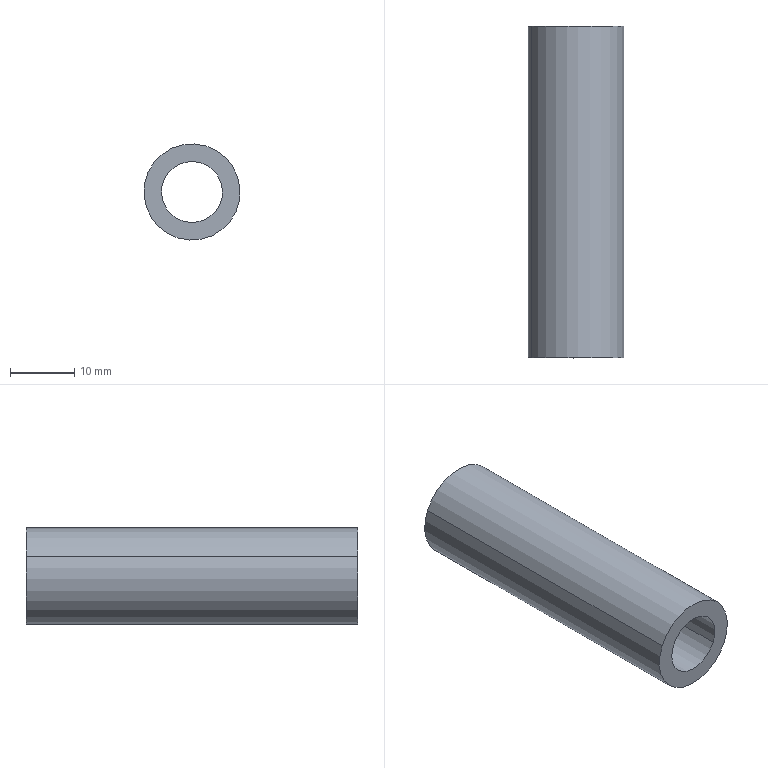Component | SolidWorks | MotorShaftHousing2-2 | 1 solid | 6 faces | box 15 x 51.75 x 15 mm | volume 5477 mm3 | cylinder 4 | plane 2 | commonest cylinder face diameters 9.5 x2 15 x2
build123d program:
from build123d import *

# Parameters (mm, degrees)
SKETCH1_R           = 7.5
SKETCH1_R_2         = 4.75
BOSS_EXTRUDE1_DEPTH = 51.75


with BuildPart() as part:
    # Sketch1 → Boss-Extrude1 (new body)
    with BuildSketch(Plane.XY):
        with Locations((-255.265, -5.179)):
            Circle(SKETCH1_R)
        with Locations((-255.265, -5.179)):
            Circle(SKETCH1_R_2, mode=Mode.SUBTRACT)
    extrude(amount=BOSS_EXTRUDE1_DEPTH)


solid = part.part

# Placed as in the assembly
solid = solid.moved(Location((218.265, 246.75, 11.179), (90, 0, 0)))
STEP:
#1=COLOUR_RGB('',0.7922,0.8196,0.9333);
#2=FILL_AREA_STYLE_COLOUR('',#1);
#3=FILL_AREA_STYLE('',(#2));
#4=SURFACE_STYLE_FILL_AREA(#3);
#5=SURFACE_SIDE_STYLE('',(#4));
#6=SURFACE_STYLE_USAGE(.BOTH.,#5);
#7=PRESENTATION_STYLE_ASSIGNMENT((#6));
#8=CARTESIAN_POINT('',(-1.628,9.715,0.3115));
#9=VERTEX_POINT('',#8);
#10=CARTESIAN_POINT('',(-1.285,9.715,0.161));
#11=VERTEX_POINT('',#10);
#12=CARTESIAN_POINT('',(-1.457,9.715,0.2362));
#13=DIRECTION('',(-0.,1.,0.));
#14=DIRECTION('',(0.9155,0.,-0.4024));
#15=AXIS2_PLACEMENT_3D('',#12,#13,#14);
#16=CIRCLE('',#15,0.187);
#17=EDGE_CURVE('',#9,#11,#16,.T.);
#18=ORIENTED_EDGE('',*,*,#17,.T.);
#19=CARTESIAN_POINT('',(-1.285,7.677,0.161));
#20=VERTEX_POINT('',#19);
#21=CARTESIAN_POINT('',(-1.285,10.55,0.161));
#22=DIRECTION('',(0.,-1.,0.));
#23=VECTOR('',#22,39.37);
#24=LINE('',#21,#23);
#25=EDGE_CURVE('',#11,#20,#24,.T.);
#26=ORIENTED_EDGE('',*,*,#25,.T.);
#27=CARTESIAN_POINT('',(-1.628,7.677,0.3115));
#28=VERTEX_POINT('',#27);
#29=CARTESIAN_POINT('',(-1.457,7.677,0.2362));
#30=DIRECTION('',(0.,1.,0.));
#31=DIRECTION('',(0.9155,0.,-0.4024));
#32=AXIS2_PLACEMENT_3D('',#29,#30,#31);
#33=CIRCLE('',#32,0.187);
#34=EDGE_CURVE('',#28,#20,#33,.T.);
#35=ORIENTED_EDGE('',*,*,#34,.F.);
#36=CARTESIAN_POINT('',(-1.628,10.55,0.3115));
#37=DIRECTION('',(0.,-1.,0.));
#38=VECTOR('',#37,39.37);
#39=LINE('',#36,#38);
#40=EDGE_CURVE('',#9,#28,#39,.T.);
#41=ORIENTED_EDGE('',*,*,#40,.F.);
#42=EDGE_LOOP('',(#18,#26,#35,#41));
#43=FACE_OUTER_BOUND('',#42,.T.);
#44=CARTESIAN_POINT('',(-1.457,10.55,0.2362));
#45=DIRECTION('',(0.,-1.,0.));
#46=DIRECTION('',(-0.9155,0.,0.4024));
#47=AXIS2_PLACEMENT_3D('',#44,#45,#46);
#48=CYLINDRICAL_SURFACE('',#47,0.187);
#49=ADVANCED_FACE('',(#43),#48,.F.);
#50=CARTESIAN_POINT('',(-1.186,9.715,0.1174));
#51=VERTEX_POINT('',#50);
#52=CARTESIAN_POINT('',(-1.727,9.715,0.355));
#53=VERTEX_POINT('',#52);
#54=CARTESIAN_POINT('',(-1.457,9.715,0.2362));
#55=DIRECTION('',(-0.,1.,0.));
#56=DIRECTION('',(0.9155,0.,-0.4024));
#57=AXIS2_PLACEMENT_3D('',#54,#55,#56);
#58=CIRCLE('',#57,0.2953);
#59=EDGE_CURVE('',#51,#53,#58,.T.);
#60=ORIENTED_EDGE('',*,*,#59,.F.);
#61=CARTESIAN_POINT('',(-1.186,7.677,0.1174));
#62=VERTEX_POINT('',#61);
#63=CARTESIAN_POINT('',(-1.186,10.55,0.1174));
#64=DIRECTION('',(0.,-1.,0.));
#65=VECTOR('',#64,39.37);
#66=LINE('',#63,#65);
#67=EDGE_CURVE('',#51,#62,#66,.T.);
#68=ORIENTED_EDGE('',*,*,#67,.T.);
#69=CARTESIAN_POINT('',(-1.727,7.677,0.355));
#70=VERTEX_POINT('',#69);
#71=CARTESIAN_POINT('',(-1.457,7.677,0.2362));
#72=DIRECTION('',(0.,1.,0.));
#73=DIRECTION('',(0.9155,0.,-0.4024));
#74=AXIS2_PLACEMENT_3D('',#71,#72,#73);
#75=CIRCLE('',#74,0.2953);
#76=EDGE_CURVE('',#62,#70,#75,.T.);
#77=ORIENTED_EDGE('',*,*,#76,.T.);
#78=CARTESIAN_POINT('',(-1.727,10.55,0.355));
#79=DIRECTION('',(0.,-1.,0.));
#80=VECTOR('',#79,39.37);
#81=LINE('',#78,#80);
#82=EDGE_CURVE('',#53,#70,#81,.T.);
#83=ORIENTED_EDGE('',*,*,#82,.F.);
#84=EDGE_LOOP('',(#60,#68,#77,#83));
#85=FACE_OUTER_BOUND('',#84,.T.);
#86=CARTESIAN_POINT('',(-1.457,10.55,0.2362));
#87=DIRECTION('',(0.,-1.,0.));
#88=DIRECTION('',(-0.9155,0.,0.4024));
#89=AXIS2_PLACEMENT_3D('',#86,#87,#88);
#90=CYLINDRICAL_SURFACE('',#89,0.2953);
#91=ADVANCED_FACE('',(#85),#90,.T.);
#92=ORIENTED_EDGE('',*,*,#67,.F.);
#93=CARTESIAN_POINT('',(-1.457,9.715,0.2362));
#94=DIRECTION('',(-0.,1.,0.));
#95=DIRECTION('',(0.9155,0.,-0.4024));
#96=AXIS2_PLACEMENT_3D('',#93,#94,#95);
#97=CIRCLE('',#96,0.2953);
#98=EDGE_CURVE('',#53,#51,#97,.T.);
#99=ORIENTED_EDGE('',*,*,#98,.F.);
#100=ORIENTED_EDGE('',*,*,#82,.T.);
#101=CARTESIAN_POINT('',(-1.457,7.677,0.2362));
#102=DIRECTION('',(0.,1.,0.));
#103=DIRECTION('',(0.9155,0.,-0.4024));
#104=AXIS2_PLACEMENT_3D('',#101,#102,#103);
#105=CIRCLE('',#104,0.2953);
#106=EDGE_CURVE('',#70,#62,#105,.T.);
#107=ORIENTED_EDGE('',*,*,#106,.T.);
#108=EDGE_LOOP('',(#92,#99,#100,#107));
#109=FACE_OUTER_BOUND('',#108,.T.);
#110=CARTESIAN_POINT('',(-1.457,10.55,0.2362));
#111=DIRECTION('',(0.,-1.,0.));
#112=DIRECTION('',(-0.9155,0.,0.4024));
#113=AXIS2_PLACEMENT_3D('',#110,#111,#112);
#114=CYLINDRICAL_SURFACE('',#113,0.2953);
#115=ADVANCED_FACE('',(#109),#114,.T.);
#116=ORIENTED_EDGE('',*,*,#106,.F.);
#117=ORIENTED_EDGE('',*,*,#76,.F.);
#118=EDGE_LOOP('',(#116,#117));
#119=FACE_OUTER_BOUND('',#118,.T.);
#120=ORIENTED_EDGE('',*,*,#34,.T.);
#121=CARTESIAN_POINT('',(-1.457,7.677,0.2362));
#122=DIRECTION('',(0.,1.,0.));
#123=DIRECTION('',(0.9155,0.,-0.4024));
#124=AXIS2_PLACEMENT_3D('',#121,#122,#123);
#125=CIRCLE('',#124,0.187);
#126=EDGE_CURVE('',#20,#28,#125,.T.);
#127=ORIENTED_EDGE('',*,*,#126,.T.);
#128=EDGE_LOOP('',(#120,#127));
#129=FACE_BOUND('',#128,.T.);
#130=CARTESIAN_POINT('',(-1.457,7.677,0.2362));
#131=DIRECTION('',(0.,1.,0.));
#132=DIRECTION('',(0.9155,0.,-0.4024));
#133=AXIS2_PLACEMENT_3D('',#130,#131,#132);
#134=PLANE('',#133);
#135=ADVANCED_FACE('',(#119,#129),#134,.F.);
#136=ORIENTED_EDGE('',*,*,#25,.F.);
#137=CARTESIAN_POINT('',(-1.457,9.715,0.2362));
#138=DIRECTION('',(-0.,1.,0.));
#139=DIRECTION('',(0.9155,0.,-0.4024));
#140=AXIS2_PLACEMENT_3D('',#137,#138,#139);
#141=CIRCLE('',#140,0.187);
#142=EDGE_CURVE('',#11,#9,#141,.T.);
#143=ORIENTED_EDGE('',*,*,#142,.T.);
#144=ORIENTED_EDGE('',*,*,#40,.T.);
#145=ORIENTED_EDGE('',*,*,#126,.F.);
#146=EDGE_LOOP('',(#136,#143,#144,#145));
#147=FACE_OUTER_BOUND('',#146,.T.);
#148=CARTESIAN_POINT('',(-1.457,10.55,0.2362));
#149=DIRECTION('',(0.,-1.,0.));
#150=DIRECTION('',(-0.9155,0.,0.4024));
#151=AXIS2_PLACEMENT_3D('',#148,#149,#150);
#152=CYLINDRICAL_SURFACE('',#151,0.187);
#153=ADVANCED_FACE('',(#147),#152,.F.);
#154=ORIENTED_EDGE('',*,*,#17,.F.);
#155=ORIENTED_EDGE('',*,*,#142,.F.);
#156=EDGE_LOOP('',(#154,#155));
#157=FACE_BOUND('',#156,.T.);
#158=ORIENTED_EDGE('',*,*,#98,.T.);
#159=ORIENTED_EDGE('',*,*,#59,.T.);
#160=EDGE_LOOP('',(#158,#159));
#161=FACE_OUTER_BOUND('',#160,.T.);
#162=CARTESIAN_POINT('',(-1.158,9.715,0.3643));
#163=DIRECTION('',(-0.,1.,0.));
#164=DIRECTION('',(-0.3942,-0.,0.919));
#165=AXIS2_PLACEMENT_3D('',#162,#163,#164);
#166=PLANE('',#165);
#167=ADVANCED_FACE('',(#157,#161),#166,.T.);
#168=CLOSED_SHELL('',(#49,#91,#115,#135,#153,#167));
#169=MANIFOLD_SOLID_BREP('',#168);
#170=STYLED_ITEM('',(#7),#169);
#171=(LENGTH_UNIT()NAMED_UNIT(*)SI_UNIT($,.METRE.));
#172=LENGTH_MEASURE_WITH_UNIT(LENGTH_MEASURE(0.0254),#171);
#173=DIMENSIONAL_EXPONENTS(1.,0.,0.,0.,0.,0.,0.);
#174=(CONVERSION_BASED_UNIT('',#172)LENGTH_UNIT()NAMED_UNIT(#173));
#175=UNCERTAINTY_MEASURE_WITH_UNIT(LENGTH_MEASURE(0.00001),#174,'','');
#176=(NAMED_UNIT(*)PLANE_ANGLE_UNIT()SI_UNIT($,.RADIAN.));
#177=(NAMED_UNIT(*)SI_UNIT($,.STERADIAN.)SOLID_ANGLE_UNIT());
#178=(GEOMETRIC_REPRESENTATION_CONTEXT(3)GLOBAL_UNCERTAINTY_ASSIGNED_CONTEXT((#175))GLOBAL_UNIT_ASSIGNED_CONTEXT((#174,#176,#177))REPRESENTATION_CONTEXT('',''));
#179=MECHANICAL_DESIGN_GEOMETRIC_PRESENTATION_REPRESENTATION('',(#170),#178);
#180=PRESENTATION_LAYER_ASSIGNMENT('','',(#170));
#181=CARTESIAN_POINT('',(0.,0.,0.));
#182=DIRECTION('',(0.,0.,1.));
#183=DIRECTION('',(1.,0.,0.));
#184=AXIS2_PLACEMENT_3D('',#181,#182,#183);
#185=(LENGTH_UNIT()NAMED_UNIT(*)SI_UNIT($,.METRE.));
#186=LENGTH_MEASURE_WITH_UNIT(LENGTH_MEASURE(0.0254),#185);
#187=DIMENSIONAL_EXPONENTS(1.,0.,0.,0.,0.,0.,0.);
#188=(CONVERSION_BASED_UNIT('',#186)LENGTH_UNIT()NAMED_UNIT(#187));
#189=UNCERTAINTY_MEASURE_WITH_UNIT(LENGTH_MEASURE(0.00001),#188,'','');
#190=(NAMED_UNIT(*)PLANE_ANGLE_UNIT()SI_UNIT($,.RADIAN.));
#191=(NAMED_UNIT(*)SI_UNIT($,.STERADIAN.)SOLID_ANGLE_UNIT());
#192=(GEOMETRIC_REPRESENTATION_CONTEXT(3)GLOBAL_UNCERTAINTY_ASSIGNED_CONTEXT((#189))GLOBAL_UNIT_ASSIGNED_CONTEXT((#188,#190,#191))REPRESENTATION_CONTEXT('',''));
#193=ADVANCED_BREP_SHAPE_REPRESENTATION('',(#169,#184),#192);